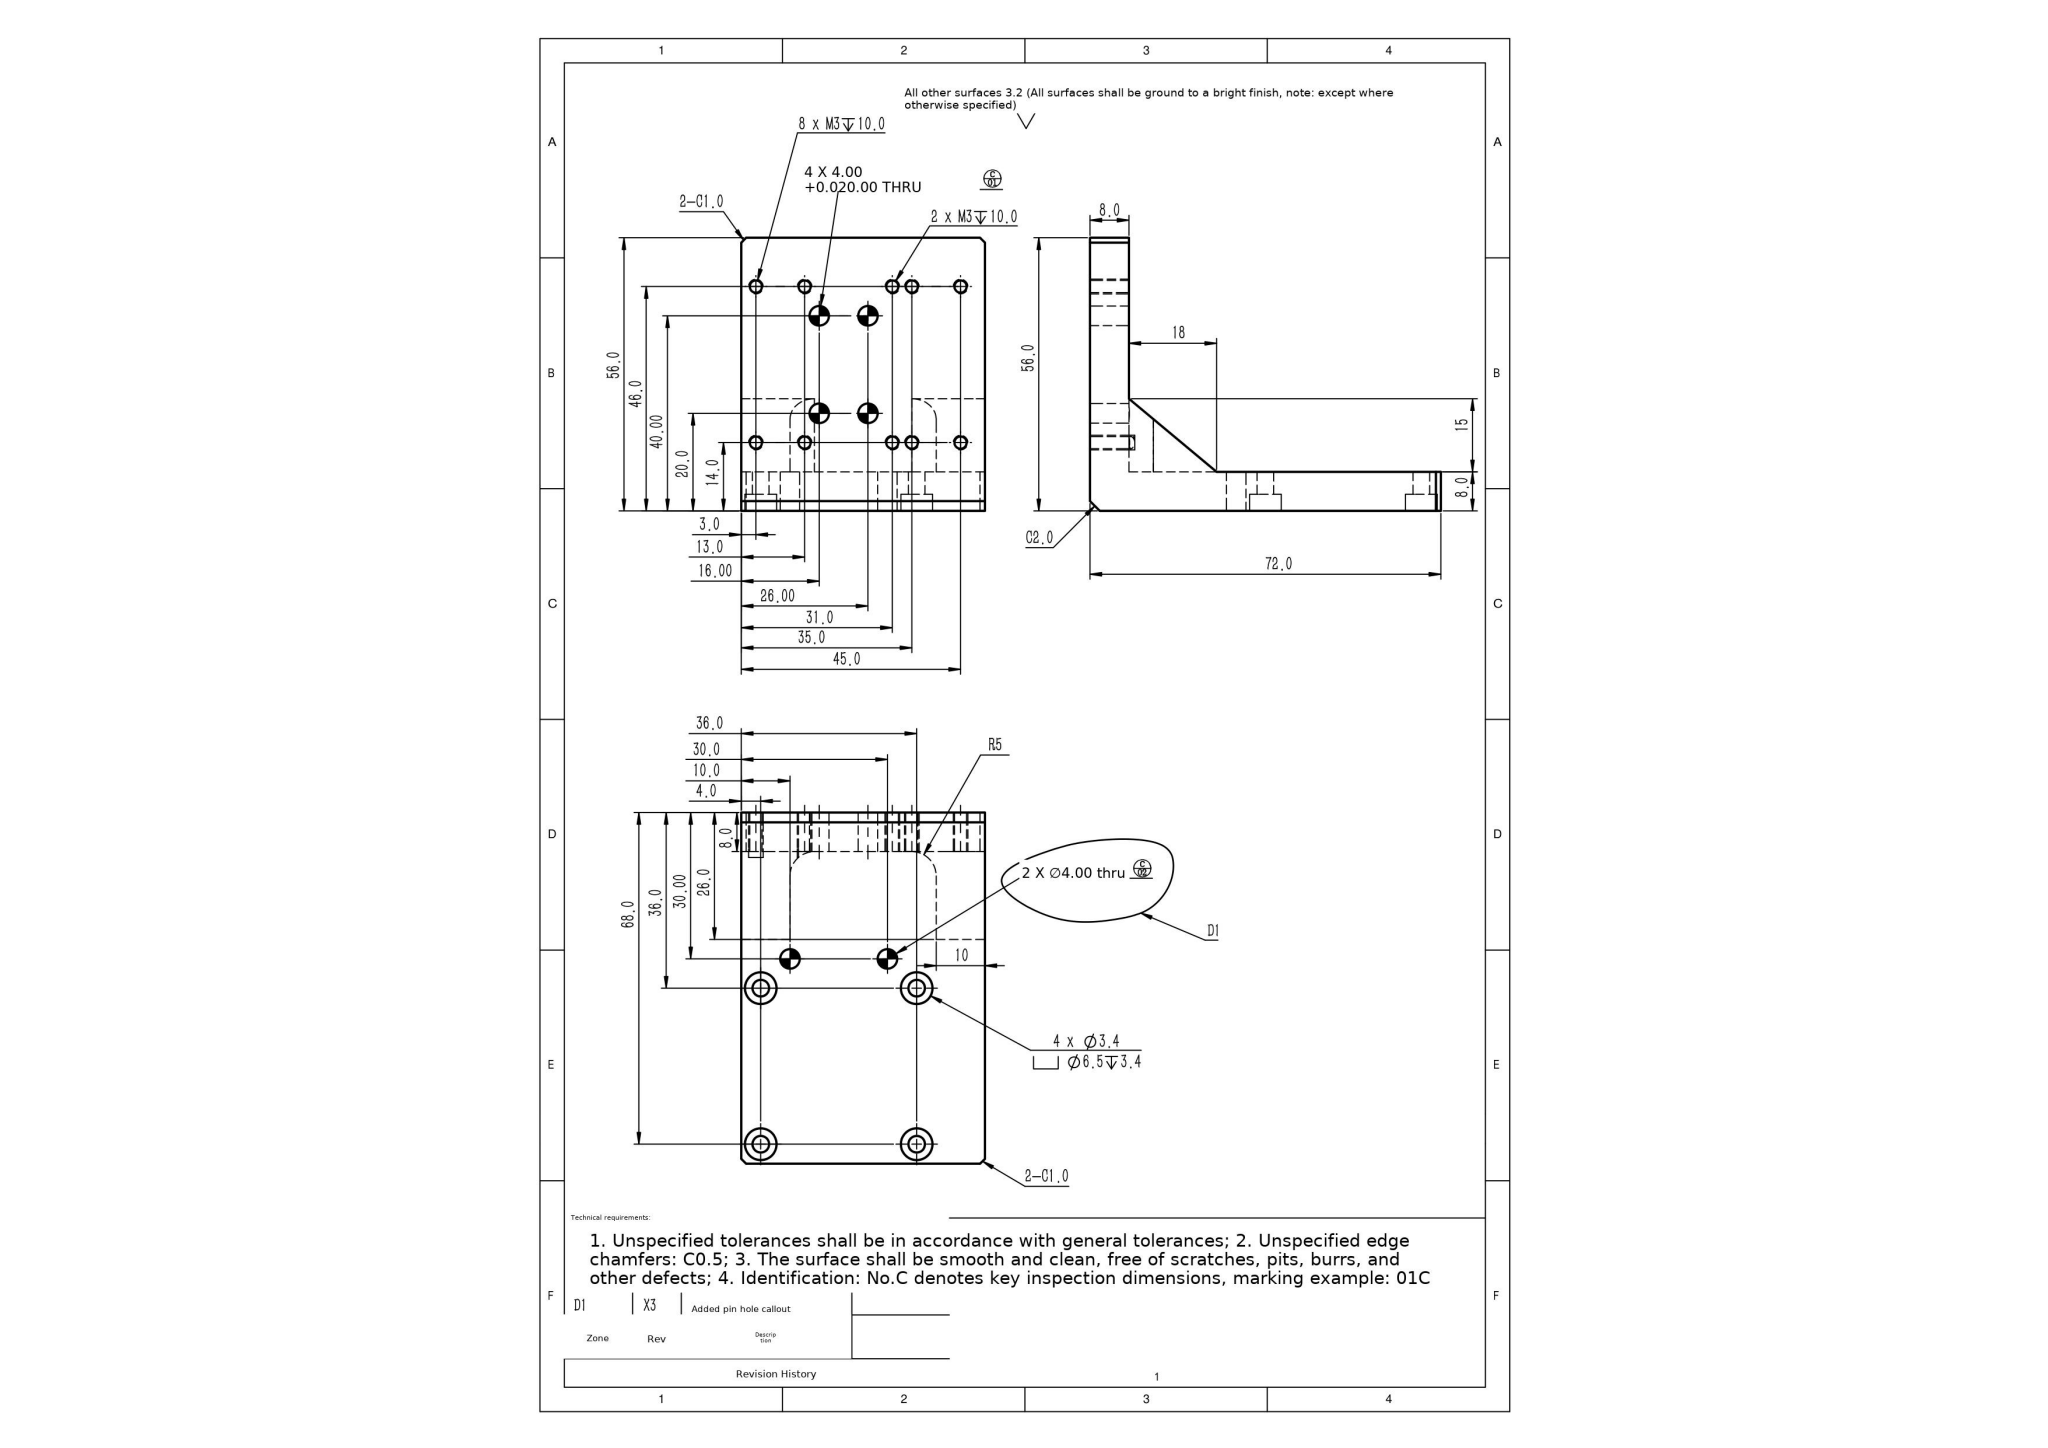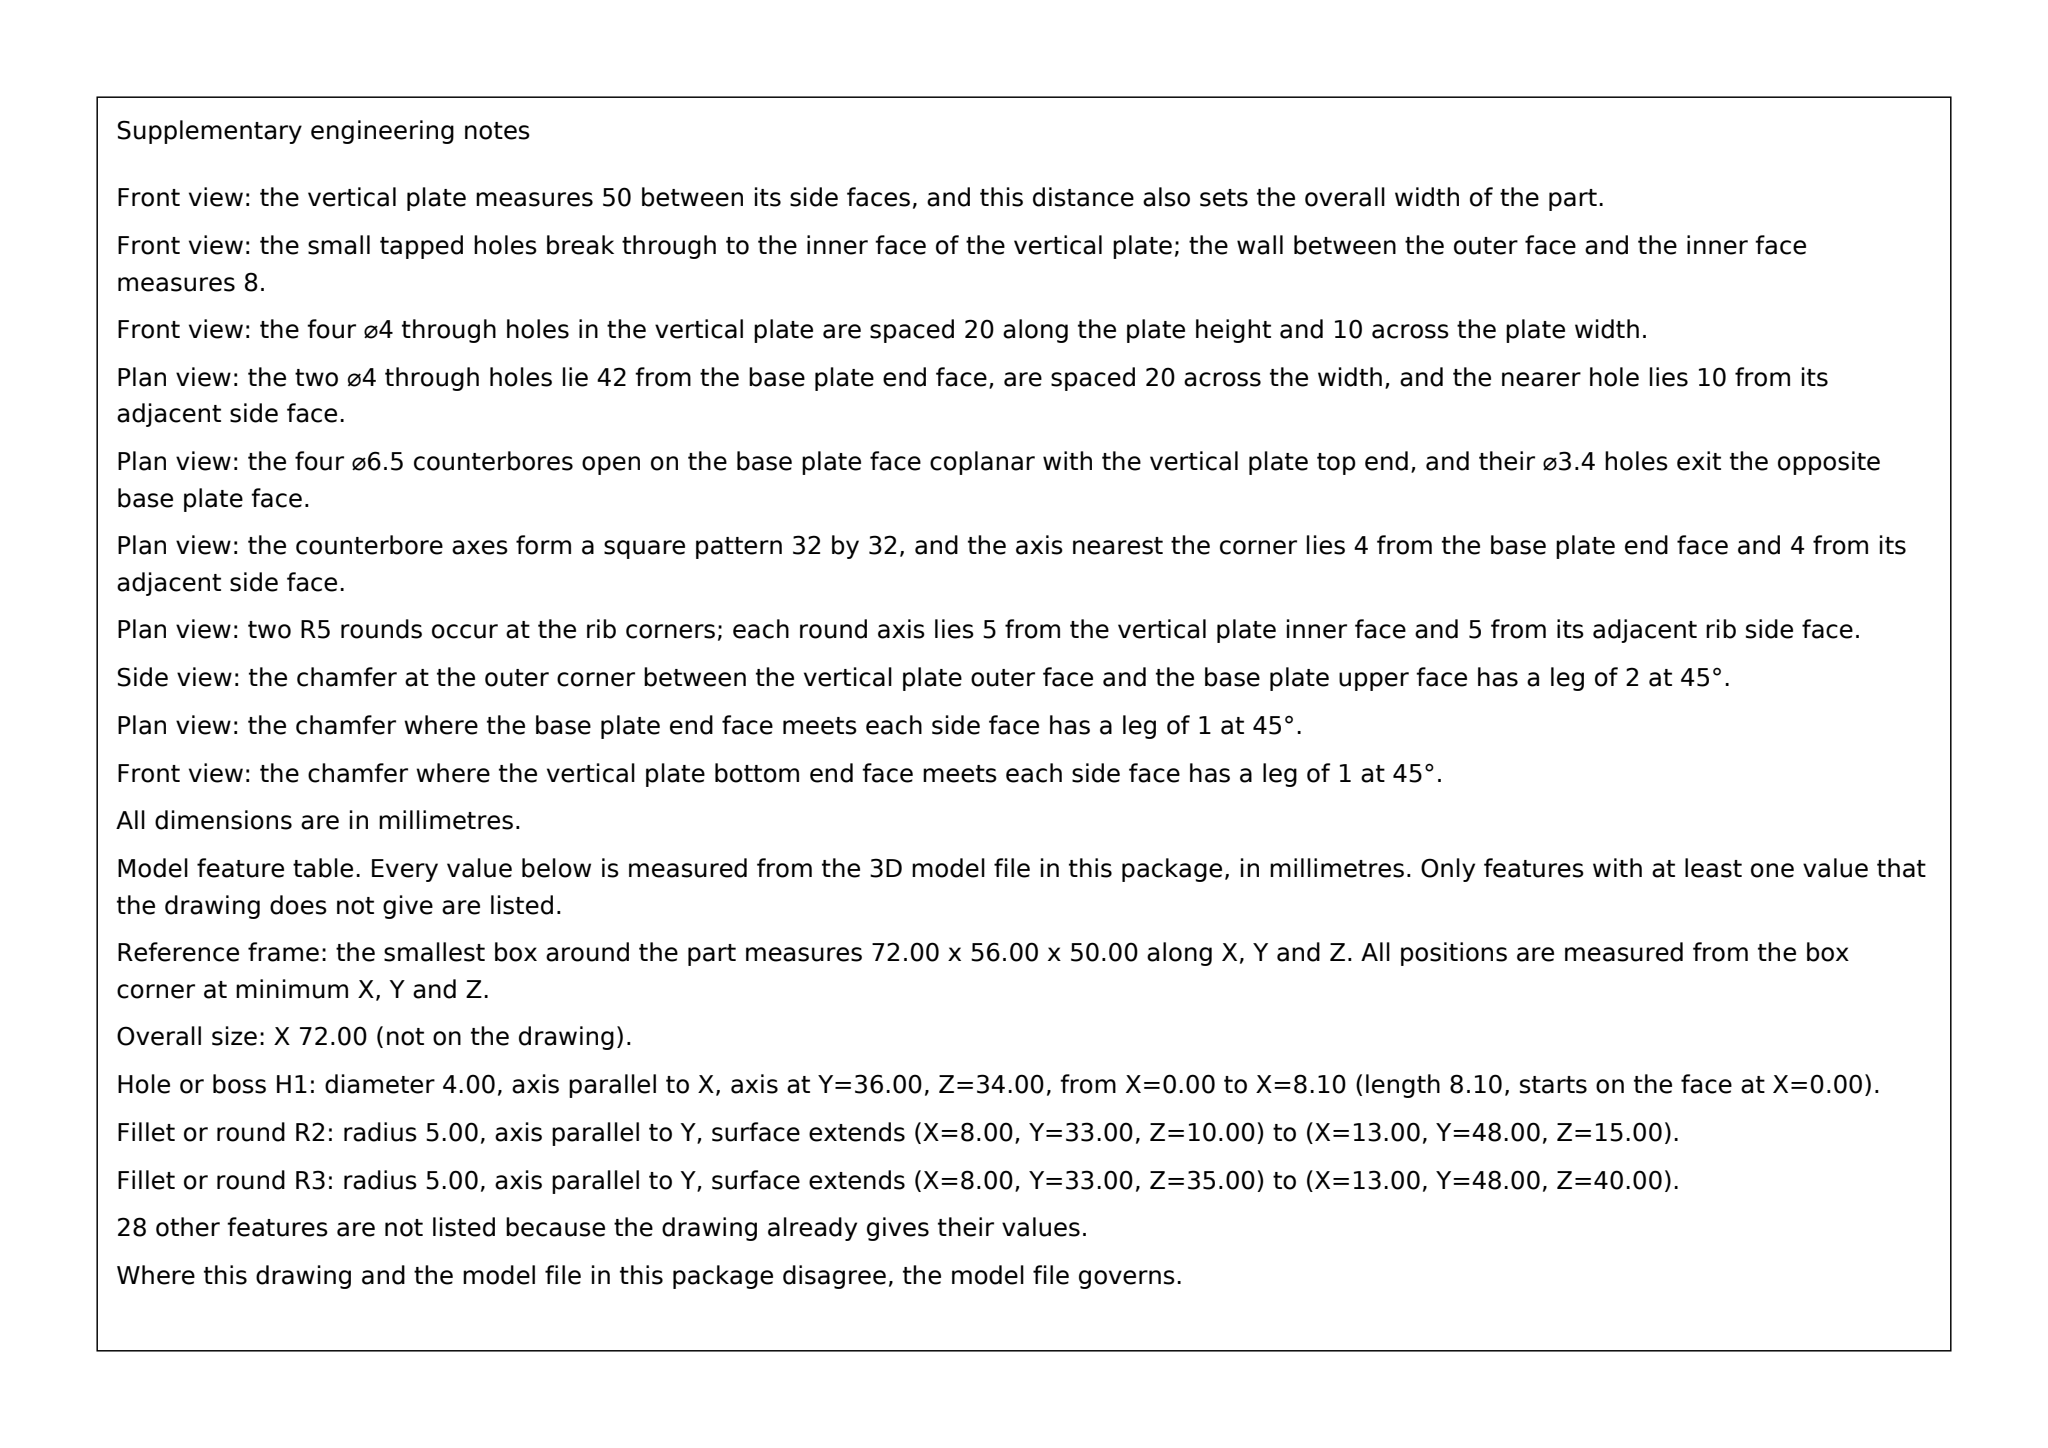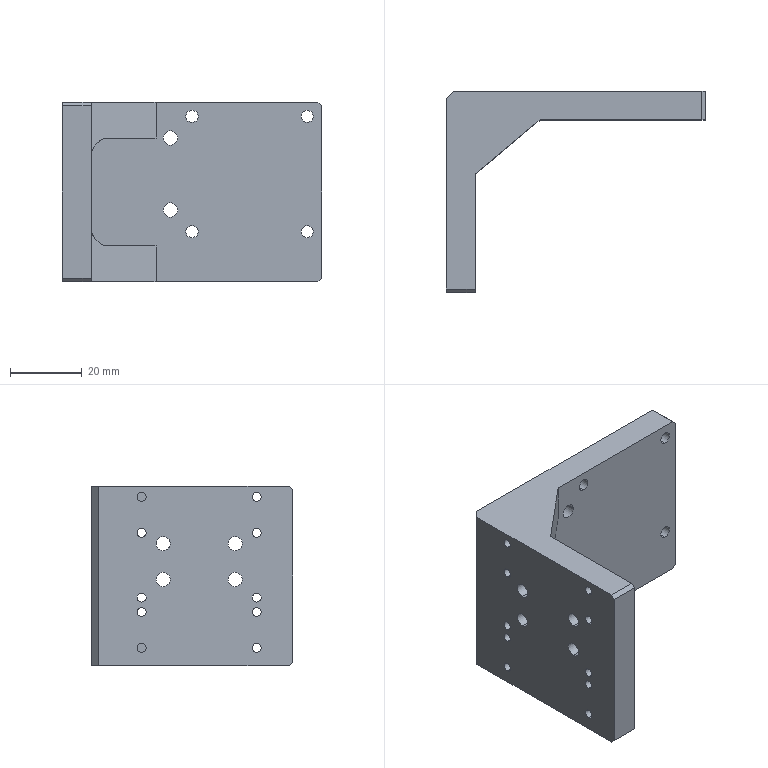Part | SolidWorks | mm | 1 solid | 73 faces | box 72 x 56 x 50 mm | volume 49118 mm3 | cylinder 50 | plane 23 | commonest cylinder face diameters 2.5 x20 4 x12 6.5 x8 3.4 x8 10 x2
Drawing notes:
RIB 30 WIDE X 15 THK, 10 FM EA SIDE EDGE | from the solid: z-planes at 10.0 and 40.0 bound rib; bbox z=50 gives 30 wide, 10 each side
GUSSET DIAG 56.3° FM BASE: 15 UP PLATE FACE TO 18 FM BACK FACE | from the solid: front face x=8, base top y=48; rise 15 over run 10 (x8->x18); atan(15/10)=56.31°
2X Ø10 DP 15 FM TOP FACE, CL 13 FM BACK FACE, 15 & 35 FM SIDE EDGE | from the solid: cyl Ø10 axis y len 15 at (x,z)=(13,15) and (13,35); back face x=0, side edge z=0
4X Ø3.4 THRU, Ø6.5 CBORE DP 3.4; CL 36 & 68 FM BACK FACE, 14 & 46 FM SIDE EDGE | from the solid: Ø3.4 len 4.6 + Ø6.5 len 3.4 axis y at (36,14),(36,46),(68,14),(68,46); plate 8 thk = thru